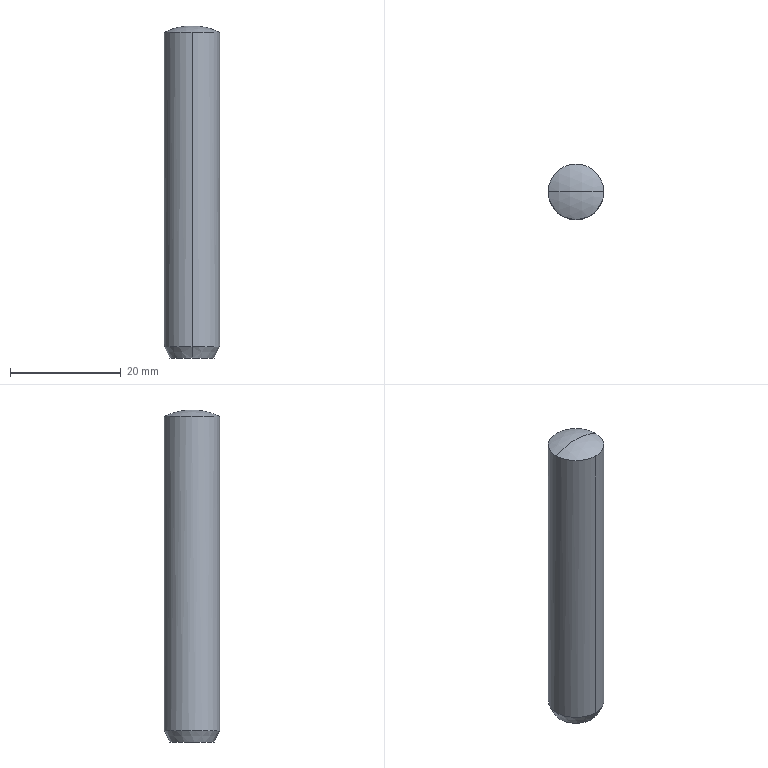Component | NX | DOWEL_PIN_10X60_2 | 1 solid | 7 faces | box 10.01 x 10.01 x 60 mm | volume 4642 mm3 | sphere 2 | cylinder 2 | cone 2 | plane 1 | commonest cylinder face diameters 10.006 x2
STEP:
#1=CARTESIAN_POINT('',(0.,0.,0.));
#2=DIRECTION('',(0.,0.,1.));
#3=DIRECTION('',(1.,0.,0.));
#4=AXIS2_PLACEMENT_3D('',#1,#2,#3);
#5=CARTESIAN_POINT('',(263.343,64.989,375.));
#6=VERTEX_POINT('',#5);
#7=CARTESIAN_POINT('',(253.337,64.989,375.));
#8=VERTEX_POINT('',#7);
#9=CARTESIAN_POINT('',(258.34,64.989,365.171));
#10=DIRECTION('',(0.,-1.,-0.));
#11=DIRECTION('',(-1.,0.,0.));
#12=AXIS2_PLACEMENT_3D('',#9,#10,#11);
#13=CIRCLE('',#12,11.029);
#14=CARTESIAN_POINT('',(258.34,64.989,365.171));
#15=DIRECTION('',(-1.,0.,0.));
#16=DIRECTION('',(0.,0.,-1.));
#17=AXIS2_PLACEMENT_3D('',#14,#15,#16);
#18=SPHERICAL_SURFACE('',#17,11.029);
#19=CARTESIAN_POINT('',(3.142,-4.712));
#20=DIRECTION('',(0.,1.));
#21=VECTOR('',#20,1.);
#22=LINE('',#19,#21);
#23=(GEOMETRIC_REPRESENTATION_CONTEXT(2)PARAMETRIC_REPRESENTATION_CONTEXT()REPRESENTATION_CONTEXT('',''));
#24=DEFINITIONAL_REPRESENTATION('',(#22),#23);
#25=PCURVE('',#18,#24);
#26=CARTESIAN_POINT('',(258.34,64.989,365.171));
#27=DIRECTION('',(-1.,0.,0.));
#28=DIRECTION('',(0.,0.,-1.));
#29=AXIS2_PLACEMENT_3D('',#26,#27,#28);
#30=SPHERICAL_SURFACE('',#29,11.029);
#31=CARTESIAN_POINT('',(3.142,-4.712));
#32=DIRECTION('',(0.,1.));
#33=VECTOR('',#32,1.);
#34=LINE('',#31,#33);
#35=(GEOMETRIC_REPRESENTATION_CONTEXT(2)PARAMETRIC_REPRESENTATION_CONTEXT()REPRESENTATION_CONTEXT('',''));
#36=DEFINITIONAL_REPRESENTATION('',(#34),#35);
#37=PCURVE('',#30,#36);
#38=SURFACE_CURVE('',#13,(#25,#37),.PCURVE_S1.);
#39=EDGE_CURVE('',#6,#8,#38,.T.);
#40=ORIENTED_EDGE('',*,*,#39,.F.);
#41=CARTESIAN_POINT('',(258.34,69.992,375.));
#42=VERTEX_POINT('',#41);
#43=CARTESIAN_POINT('',(258.34,64.989,375.));
#44=DIRECTION('',(0.,0.,1.));
#45=DIRECTION('',(0.,1.,0.));
#46=AXIS2_PLACEMENT_3D('',#43,#44,#45);
#47=CIRCLE('',#46,5.003);
#48=CARTESIAN_POINT('',(3.142,-0.4708));
#49=CARTESIAN_POINT('',(3.154,-0.4708));
#50=CARTESIAN_POINT('',(3.178,-0.47));
#51=CARTESIAN_POINT('',(3.214,-0.4661));
#52=CARTESIAN_POINT('',(3.25,-0.4596));
#53=CARTESIAN_POINT('',(3.284,-0.4507));
#54=CARTESIAN_POINT('',(3.318,-0.4394));
#55=CARTESIAN_POINT('',(3.35,-0.4257));
#56=CARTESIAN_POINT('',(3.381,-0.4098));
#57=CARTESIAN_POINT('',(3.41,-0.3919));
#58=CARTESIAN_POINT('',(3.438,-0.3719));
#59=CARTESIAN_POINT('',(3.464,-0.3502));
#60=CARTESIAN_POINT('',(3.487,-0.3268));
#61=CARTESIAN_POINT('',(3.509,-0.3018));
#62=CARTESIAN_POINT('',(3.529,-0.2755));
#63=CARTESIAN_POINT('',(3.547,-0.248));
#64=CARTESIAN_POINT('',(3.562,-0.2193));
#65=CARTESIAN_POINT('',(3.576,-0.1897));
#66=CARTESIAN_POINT('',(3.587,-0.1593));
#67=CARTESIAN_POINT('',(3.596,-0.1282));
#68=CARTESIAN_POINT('',(3.603,-0.09664));
#69=CARTESIAN_POINT('',(3.609,-0.06464));
#70=CARTESIAN_POINT('',(3.612,-0.03239));
#71=CARTESIAN_POINT('',(3.612,-0.0108));
#72=CARTESIAN_POINT('',(3.612,0.));
#73=B_SPLINE_CURVE_WITH_KNOTS('',3,(#48,#49,#50,#51,#52,#53,#54,#55,#56,#57,#58,#59,#60,#61,#62,#63,#64,#65,#66,#67,#68,#69,#70,#71,#72),.UNSPECIFIED.,.F.,.F.,(4,1,1,1,1,1,1,1,1,1,1,1,1,1,1,1,1,1,1,1,1,1,4),(4.712,4.784,4.855,4.927,4.998,5.069,5.141,5.212,5.284,5.355,5.426,5.498,5.569,5.641,5.712,5.783,5.855,5.926,5.998,6.069,6.14,6.212,6.283),.QUASI_UNIFORM_KNOTS.);
#74=(GEOMETRIC_REPRESENTATION_CONTEXT(2)PARAMETRIC_REPRESENTATION_CONTEXT()REPRESENTATION_CONTEXT('',''));
#75=DEFINITIONAL_REPRESENTATION('',(#73),#74);
#76=PCURVE('',#18,#75);
#77=CARTESIAN_POINT('',(258.34,64.989,336.601));
#78=DIRECTION('',(0.,0.,1.));
#79=DIRECTION('',(0.,-1.,0.));
#80=AXIS2_PLACEMENT_3D('',#77,#78,#79);
#81=CYLINDRICAL_SURFACE('',#80,5.003);
#82=CARTESIAN_POINT('',(-3.142,38.399));
#83=DIRECTION('',(1.,0.));
#84=VECTOR('',#83,1.);
#85=LINE('',#82,#84);
#86=(GEOMETRIC_REPRESENTATION_CONTEXT(2)PARAMETRIC_REPRESENTATION_CONTEXT()REPRESENTATION_CONTEXT('',''));
#87=DEFINITIONAL_REPRESENTATION('',(#85),#86);
#88=PCURVE('',#81,#87);
#89=SURFACE_CURVE('',#47,(#76,#88),.PCURVE_S1.);
#90=EDGE_CURVE('',#6,#42,#89,.T.);
#91=ORIENTED_EDGE('',*,*,#90,.T.);
#92=CARTESIAN_POINT('',(258.34,64.989,375.));
#93=DIRECTION('',(0.,0.,1.));
#94=DIRECTION('',(0.,1.,0.));
#95=AXIS2_PLACEMENT_3D('',#92,#93,#94);
#96=CIRCLE('',#95,5.003);
#97=CARTESIAN_POINT('',(3.612,0.));
#98=CARTESIAN_POINT('',(3.612,0.0108));
#99=CARTESIAN_POINT('',(3.612,0.03239));
#100=CARTESIAN_POINT('',(3.609,0.06464));
#101=CARTESIAN_POINT('',(3.603,0.09664));
#102=CARTESIAN_POINT('',(3.596,0.1282));
#103=CARTESIAN_POINT('',(3.587,0.1593));
#104=CARTESIAN_POINT('',(3.576,0.1897));
#105=CARTESIAN_POINT('',(3.562,0.2193));
#106=CARTESIAN_POINT('',(3.547,0.248));
#107=CARTESIAN_POINT('',(3.529,0.2755));
#108=CARTESIAN_POINT('',(3.509,0.3018));
#109=CARTESIAN_POINT('',(3.487,0.3268));
#110=CARTESIAN_POINT('',(3.464,0.3502));
#111=CARTESIAN_POINT('',(3.438,0.3719));
#112=CARTESIAN_POINT('',(3.41,0.3919));
#113=CARTESIAN_POINT('',(3.381,0.4098));
#114=CARTESIAN_POINT('',(3.35,0.4257));
#115=CARTESIAN_POINT('',(3.318,0.4394));
#116=CARTESIAN_POINT('',(3.284,0.4507));
#117=CARTESIAN_POINT('',(3.25,0.4596));
#118=CARTESIAN_POINT('',(3.214,0.4661));
#119=CARTESIAN_POINT('',(3.178,0.47));
#120=CARTESIAN_POINT('',(3.154,0.4708));
#121=CARTESIAN_POINT('',(3.142,0.4708));
#122=B_SPLINE_CURVE_WITH_KNOTS('',3,(#97,#98,#99,#100,#101,#102,#103,#104,#105,#106,#107,#108,#109,#110,#111,#112,#113,#114,#115,#116,#117,#118,#119,#120,#121),.UNSPECIFIED.,.F.,.F.,(4,1,1,1,1,1,1,1,1,1,1,1,1,1,1,1,1,1,1,1,1,1,4),(0.,0.0714,0.1428,0.2142,0.2856,0.357,0.4284,0.4998,0.5712,0.6426,0.714,0.7854,0.8568,0.9282,0.9996,1.071,1.142,1.214,1.285,1.357,1.428,1.499,1.571),.QUASI_UNIFORM_KNOTS.);
#123=(GEOMETRIC_REPRESENTATION_CONTEXT(2)PARAMETRIC_REPRESENTATION_CONTEXT()REPRESENTATION_CONTEXT('',''));
#124=DEFINITIONAL_REPRESENTATION('',(#122),#123);
#125=PCURVE('',#18,#124);
#126=CARTESIAN_POINT('',(258.34,64.989,336.601));
#127=DIRECTION('',(0.,0.,1.));
#128=DIRECTION('',(0.,-1.,0.));
#129=AXIS2_PLACEMENT_3D('',#126,#127,#128);
#130=CYLINDRICAL_SURFACE('',#129,5.003);
#131=CARTESIAN_POINT('',(3.142,38.399));
#132=DIRECTION('',(1.,0.));
#133=VECTOR('',#132,1.);
#134=LINE('',#131,#133);
#135=(GEOMETRIC_REPRESENTATION_CONTEXT(2)PARAMETRIC_REPRESENTATION_CONTEXT()REPRESENTATION_CONTEXT('',''));
#136=DEFINITIONAL_REPRESENTATION('',(#134),#135);
#137=PCURVE('',#130,#136);
#138=SURFACE_CURVE('',#96,(#125,#137),.PCURVE_S1.);
#139=EDGE_CURVE('',#42,#8,#138,.T.);
#140=ORIENTED_EDGE('',*,*,#139,.T.);
#141=EDGE_LOOP('',(#40,#91,#140));
#142=FACE_BOUND('',#141,.T.);
#143=ADVANCED_FACE('',(#142),#18,.T.);
#144=CARTESIAN_POINT('',(258.34,69.992,318.201));
#145=VERTEX_POINT('',#144);
#146=CARTESIAN_POINT('',(258.34,69.992,336.601));
#147=DIRECTION('',(0.,0.,1.));
#148=VECTOR('',#147,1.);
#149=LINE('',#146,#148);
#150=CARTESIAN_POINT('',(3.142,0.));
#151=DIRECTION('',(0.,1.));
#152=VECTOR('',#151,1.);
#153=LINE('',#150,#152);
#154=(GEOMETRIC_REPRESENTATION_CONTEXT(2)PARAMETRIC_REPRESENTATION_CONTEXT()REPRESENTATION_CONTEXT('',''));
#155=DEFINITIONAL_REPRESENTATION('',(#153),#154);
#156=PCURVE('',#130,#155);
#157=CARTESIAN_POINT('',(3.142,0.));
#158=DIRECTION('',(0.,1.));
#159=VECTOR('',#158,1.);
#160=LINE('',#157,#159);
#161=(GEOMETRIC_REPRESENTATION_CONTEXT(2)PARAMETRIC_REPRESENTATION_CONTEXT()REPRESENTATION_CONTEXT('',''));
#162=DEFINITIONAL_REPRESENTATION('',(#160),#161);
#163=PCURVE('',#81,#162);
#164=SURFACE_CURVE('',#149,(#156,#163),.PCURVE_S1.);
#165=EDGE_CURVE('',#145,#42,#164,.T.);
#166=ORIENTED_EDGE('',*,*,#165,.F.);
#167=CARTESIAN_POINT('',(258.34,59.986,318.201));
#168=VERTEX_POINT('',#167);
#169=CARTESIAN_POINT('',(258.34,64.989,318.201));
#170=DIRECTION('',(0.,0.,1.));
#171=DIRECTION('',(0.,1.,0.));
#172=AXIS2_PLACEMENT_3D('',#169,#170,#171);
#173=CIRCLE('',#172,5.003);
#174=CARTESIAN_POINT('',(3.142,-18.399));
#175=DIRECTION('',(1.,0.));
#176=VECTOR('',#175,1.);
#177=LINE('',#174,#176);
#178=(GEOMETRIC_REPRESENTATION_CONTEXT(2)PARAMETRIC_REPRESENTATION_CONTEXT()REPRESENTATION_CONTEXT('',''));
#179=DEFINITIONAL_REPRESENTATION('',(#177),#178);
#180=PCURVE('',#130,#179);
#181=CARTESIAN_POINT('',(258.34,64.989,317.201));
#182=DIRECTION('',(0.,0.,1.));
#183=DIRECTION('',(0.,-1.,0.));
#184=AXIS2_PLACEMENT_3D('',#181,#182,#183);
#185=CONICAL_SURFACE('',#184,4.503,0.4636);
#186=CARTESIAN_POINT('',(3.142,1.001));
#187=DIRECTION('',(1.,0.));
#188=VECTOR('',#187,1.);
#189=LINE('',#186,#188);
#190=(GEOMETRIC_REPRESENTATION_CONTEXT(2)PARAMETRIC_REPRESENTATION_CONTEXT()REPRESENTATION_CONTEXT('',''));
#191=DEFINITIONAL_REPRESENTATION('',(#189),#190);
#192=PCURVE('',#185,#191);
#193=SURFACE_CURVE('',#173,(#180,#192),.PCURVE_S1.);
#194=EDGE_CURVE('',#145,#168,#193,.T.);
#195=ORIENTED_EDGE('',*,*,#194,.T.);
#196=CARTESIAN_POINT('',(258.34,59.986,375.));
#197=VERTEX_POINT('',#196);
#198=CARTESIAN_POINT('',(258.34,59.986,336.601));
#199=DIRECTION('',(0.,0.,-1.));
#200=VECTOR('',#199,1.);
#201=LINE('',#198,#200);
#202=CARTESIAN_POINT('',(6.283,0.));
#203=DIRECTION('',(0.,-1.));
#204=VECTOR('',#203,1.);
#205=LINE('',#202,#204);
#206=(GEOMETRIC_REPRESENTATION_CONTEXT(2)PARAMETRIC_REPRESENTATION_CONTEXT()REPRESENTATION_CONTEXT('',''));
#207=DEFINITIONAL_REPRESENTATION('',(#205),#206);
#208=PCURVE('',#130,#207);
#209=CARTESIAN_POINT('',(0.,0.));
#210=DIRECTION('',(0.,-1.));
#211=VECTOR('',#210,1.);
#212=LINE('',#209,#211);
#213=(GEOMETRIC_REPRESENTATION_CONTEXT(2)PARAMETRIC_REPRESENTATION_CONTEXT()REPRESENTATION_CONTEXT('',''));
#214=DEFINITIONAL_REPRESENTATION('',(#212),#213);
#215=PCURVE('',#81,#214);
#216=SURFACE_CURVE('',#201,(#208,#215),.PCURVE_S1.);
#217=EDGE_CURVE('',#197,#168,#216,.T.);
#218=ORIENTED_EDGE('',*,*,#217,.F.);
#219=CARTESIAN_POINT('',(258.34,64.989,375.));
#220=DIRECTION('',(0.,0.,1.));
#221=DIRECTION('',(0.,1.,0.));
#222=AXIS2_PLACEMENT_3D('',#219,#220,#221);
#223=CIRCLE('',#222,5.003);
#224=CARTESIAN_POINT('',(3.142,38.399));
#225=DIRECTION('',(1.,0.));
#226=VECTOR('',#225,1.);
#227=LINE('',#224,#226);
#228=(GEOMETRIC_REPRESENTATION_CONTEXT(2)PARAMETRIC_REPRESENTATION_CONTEXT()REPRESENTATION_CONTEXT('',''));
#229=DEFINITIONAL_REPRESENTATION('',(#227),#228);
#230=PCURVE('',#130,#229);
#231=CARTESIAN_POINT('',(3.142,0.4708));
#232=CARTESIAN_POINT('',(3.129,0.4708));
#233=CARTESIAN_POINT('',(3.105,0.47));
#234=CARTESIAN_POINT('',(3.069,0.4661));
#235=CARTESIAN_POINT('',(3.034,0.4596));
#236=CARTESIAN_POINT('',(2.999,0.4507));
#237=CARTESIAN_POINT('',(2.965,0.4394));
#238=CARTESIAN_POINT('',(2.933,0.4257));
#239=CARTESIAN_POINT('',(2.902,0.4098));
#240=CARTESIAN_POINT('',(2.873,0.3919));
#241=CARTESIAN_POINT('',(2.845,0.3719));
#242=CARTESIAN_POINT('',(2.82,0.3502));
#243=CARTESIAN_POINT('',(2.796,0.3268));
#244=CARTESIAN_POINT('',(2.774,0.3018));
#245=CARTESIAN_POINT('',(2.754,0.2755));
#246=CARTESIAN_POINT('',(2.737,0.248));
#247=CARTESIAN_POINT('',(2.721,0.2193));
#248=CARTESIAN_POINT('',(2.708,0.1897));
#249=CARTESIAN_POINT('',(2.696,0.1593));
#250=CARTESIAN_POINT('',(2.687,0.1282));
#251=CARTESIAN_POINT('',(2.68,0.09664));
#252=CARTESIAN_POINT('',(2.675,0.06464));
#253=CARTESIAN_POINT('',(2.671,0.03239));
#254=CARTESIAN_POINT('',(2.671,0.0108));
#255=CARTESIAN_POINT('',(2.671,0.));
#256=B_SPLINE_CURVE_WITH_KNOTS('',3,(#231,#232,#233,#234,#235,#236,#237,#238,#239,#240,#241,#242,#243,#244,#245,#246,#247,#248,#249,#250,#251,#252,#253,#254,#255),.UNSPECIFIED.,.F.,.F.,(4,1,1,1,1,1,1,1,1,1,1,1,1,1,1,1,1,1,1,1,1,1,4),(1.571,1.642,1.714,1.785,1.856,1.928,1.999,2.071,2.142,2.213,2.285,2.356,2.428,2.499,2.57,2.642,2.713,2.785,2.856,2.927,2.999,3.07,3.142),.QUASI_UNIFORM_KNOTS.);
#257=(GEOMETRIC_REPRESENTATION_CONTEXT(2)PARAMETRIC_REPRESENTATION_CONTEXT()REPRESENTATION_CONTEXT('',''));
#258=DEFINITIONAL_REPRESENTATION('',(#256),#257);
#259=PCURVE('',#30,#258);
#260=SURFACE_CURVE('',#223,(#230,#259),.PCURVE_S1.);
#261=EDGE_CURVE('',#8,#197,#260,.T.);
#262=ORIENTED_EDGE('',*,*,#261,.F.);
#263=ORIENTED_EDGE('',*,*,#139,.F.);
#264=EDGE_LOOP('',(#166,#195,#218,#262,#263));
#265=FACE_BOUND('',#264,.T.);
#266=ADVANCED_FACE('',(#265),#130,.T.);
#267=CARTESIAN_POINT('',(258.34,68.991,316.2));
#268=VERTEX_POINT('',#267);
#269=CARTESIAN_POINT('',(258.34,69.491,317.201));
#270=DIRECTION('',(0.,0.4472,0.8944));
#271=VECTOR('',#270,1.);
#272=LINE('',#269,#271);
#273=CARTESIAN_POINT('',(3.142,-0.));
#274=DIRECTION('',(0.,1.));
#275=VECTOR('',#274,1.);
#276=LINE('',#273,#275);
#277=(GEOMETRIC_REPRESENTATION_CONTEXT(2)PARAMETRIC_REPRESENTATION_CONTEXT()REPRESENTATION_CONTEXT('',''));
#278=DEFINITIONAL_REPRESENTATION('',(#276),#277);
#279=PCURVE('',#185,#278);
#280=CARTESIAN_POINT('',(258.34,64.989,317.201));
#281=DIRECTION('',(0.,0.,1.));
#282=DIRECTION('',(0.,-1.,0.));
#283=AXIS2_PLACEMENT_3D('',#280,#281,#282);
#284=CONICAL_SURFACE('',#283,4.503,0.4636);
#285=CARTESIAN_POINT('',(3.142,-0.));
#286=DIRECTION('',(0.,1.));
#287=VECTOR('',#286,1.);
#288=LINE('',#285,#287);
#289=(GEOMETRIC_REPRESENTATION_CONTEXT(2)PARAMETRIC_REPRESENTATION_CONTEXT()REPRESENTATION_CONTEXT('',''));
#290=DEFINITIONAL_REPRESENTATION('',(#288),#289);
#291=PCURVE('',#284,#290);
#292=SURFACE_CURVE('',#272,(#279,#291),.PCURVE_S1.);
#293=EDGE_CURVE('',#268,#145,#292,.T.);
#294=ORIENTED_EDGE('',*,*,#293,.F.);
#295=CARTESIAN_POINT('',(258.34,60.986,316.2));
#296=VERTEX_POINT('',#295);
#297=CARTESIAN_POINT('',(258.34,64.989,316.2));
#298=DIRECTION('',(0.,0.,1.));
#299=DIRECTION('',(0.,1.,0.));
#300=AXIS2_PLACEMENT_3D('',#297,#298,#299);
#301=CIRCLE('',#300,4.002);
#302=CARTESIAN_POINT('',(3.142,-1.001));
#303=DIRECTION('',(1.,0.));
#304=VECTOR('',#303,1.);
#305=LINE('',#302,#304);
#306=(GEOMETRIC_REPRESENTATION_CONTEXT(2)PARAMETRIC_REPRESENTATION_CONTEXT()REPRESENTATION_CONTEXT('',''));
#307=DEFINITIONAL_REPRESENTATION('',(#305),#306);
#308=PCURVE('',#185,#307);
#309=CARTESIAN_POINT('',(258.34,66.99,316.2));
#310=DIRECTION('',(0.,-0.,-1.));
#311=DIRECTION('',(0.,1.,-0.));
#312=AXIS2_PLACEMENT_3D('',#309,#310,#311);
#313=PLANE('',#312);
#314=CARTESIAN_POINT('',(2.001,0.));
#315=CARTESIAN_POINT('',(2.001,-6.932));
#316=CARTESIAN_POINT('',(-4.002,-3.466));
#317=CARTESIAN_POINT('',(-10.006,-0.));
#318=CARTESIAN_POINT('',(-4.002,3.466));
#319=CARTESIAN_POINT('',(2.001,6.932));
#320=CARTESIAN_POINT('',(2.001,0.));
#321=(BOUNDED_CURVE()B_SPLINE_CURVE(2,(#314,#315,#316,#317,#318,#319,#320),.UNSPECIFIED.,.T.,.F.)B_SPLINE_CURVE_WITH_KNOTS((1,2,2,2,2,1),(-2.094,0.,2.094,4.189,6.283,8.378),.UNSPECIFIED.)CURVE()GEOMETRIC_REPRESENTATION_ITEM()RATIONAL_B_SPLINE_CURVE((1.,0.5,1.,0.5,1.,0.5,1.))REPRESENTATION_ITEM(''));
#322=(GEOMETRIC_REPRESENTATION_CONTEXT(2)PARAMETRIC_REPRESENTATION_CONTEXT()REPRESENTATION_CONTEXT('',''));
#323=DEFINITIONAL_REPRESENTATION('',(#321),#322);
#324=PCURVE('',#313,#323);
#325=SURFACE_CURVE('',#301,(#308,#324),.PCURVE_S1.);
#326=EDGE_CURVE('',#268,#296,#325,.T.);
#327=ORIENTED_EDGE('',*,*,#326,.T.);
#328=CARTESIAN_POINT('',(258.34,60.486,317.201));
#329=DIRECTION('',(0.,0.4472,-0.8944));
#330=VECTOR('',#329,1.);
#331=LINE('',#328,#330);
#332=CARTESIAN_POINT('',(6.283,-0.));
#333=DIRECTION('',(0.,-1.));
#334=VECTOR('',#333,1.);
#335=LINE('',#332,#334);
#336=(GEOMETRIC_REPRESENTATION_CONTEXT(2)PARAMETRIC_REPRESENTATION_CONTEXT()REPRESENTATION_CONTEXT('',''));
#337=DEFINITIONAL_REPRESENTATION('',(#335),#336);
#338=PCURVE('',#185,#337);
#339=CARTESIAN_POINT('',(0.,-0.));
#340=DIRECTION('',(0.,-1.));
#341=VECTOR('',#340,1.);
#342=LINE('',#339,#341);
#343=(GEOMETRIC_REPRESENTATION_CONTEXT(2)PARAMETRIC_REPRESENTATION_CONTEXT()REPRESENTATION_CONTEXT('',''));
#344=DEFINITIONAL_REPRESENTATION('',(#342),#343);
#345=PCURVE('',#284,#344);
#346=SURFACE_CURVE('',#331,(#338,#345),.PCURVE_S1.);
#347=EDGE_CURVE('',#168,#296,#346,.T.);
#348=ORIENTED_EDGE('',*,*,#347,.F.);
#349=ORIENTED_EDGE('',*,*,#194,.F.);
#350=EDGE_LOOP('',(#294,#327,#348,#349));
#351=FACE_BOUND('',#350,.T.);
#352=ADVANCED_FACE('',(#351),#185,.T.);
#353=ORIENTED_EDGE('',*,*,#293,.T.);
#354=CARTESIAN_POINT('',(258.34,64.989,318.201));
#355=DIRECTION('',(0.,0.,1.));
#356=DIRECTION('',(0.,1.,0.));
#357=AXIS2_PLACEMENT_3D('',#354,#355,#356);
#358=CIRCLE('',#357,5.003);
#359=CARTESIAN_POINT('',(-3.142,1.001));
#360=DIRECTION('',(1.,0.));
#361=VECTOR('',#360,1.);
#362=LINE('',#359,#361);
#363=(GEOMETRIC_REPRESENTATION_CONTEXT(2)PARAMETRIC_REPRESENTATION_CONTEXT()REPRESENTATION_CONTEXT('',''));
#364=DEFINITIONAL_REPRESENTATION('',(#362),#363);
#365=PCURVE('',#284,#364);
#366=CARTESIAN_POINT('',(-3.142,-18.399));
#367=DIRECTION('',(1.,0.));
#368=VECTOR('',#367,1.);
#369=LINE('',#366,#368);
#370=(GEOMETRIC_REPRESENTATION_CONTEXT(2)PARAMETRIC_REPRESENTATION_CONTEXT()REPRESENTATION_CONTEXT('',''));
#371=DEFINITIONAL_REPRESENTATION('',(#369),#370);
#372=PCURVE('',#81,#371);
#373=SURFACE_CURVE('',#358,(#365,#372),.PCURVE_S1.);
#374=EDGE_CURVE('',#168,#145,#373,.T.);
#375=ORIENTED_EDGE('',*,*,#374,.F.);
#376=ORIENTED_EDGE('',*,*,#347,.T.);
#377=CARTESIAN_POINT('',(258.34,64.989,316.2));
#378=DIRECTION('',(0.,0.,1.));
#379=DIRECTION('',(0.,1.,0.));
#380=AXIS2_PLACEMENT_3D('',#377,#378,#379);
#381=CIRCLE('',#380,4.002);
#382=CARTESIAN_POINT('',(-3.142,-1.001));
#383=DIRECTION('',(1.,-0.));
#384=VECTOR('',#383,1.);
#385=LINE('',#382,#384);
#386=(GEOMETRIC_REPRESENTATION_CONTEXT(2)PARAMETRIC_REPRESENTATION_CONTEXT()REPRESENTATION_CONTEXT('',''));
#387=DEFINITIONAL_REPRESENTATION('',(#385),#386);
#388=PCURVE('',#284,#387);
#389=CARTESIAN_POINT('',(2.001,0.));
#390=CARTESIAN_POINT('',(2.001,-6.932));
#391=CARTESIAN_POINT('',(-4.002,-3.466));
#392=CARTESIAN_POINT('',(-10.006,-0.));
#393=CARTESIAN_POINT('',(-4.002,3.466));
#394=CARTESIAN_POINT('',(2.001,6.932));
#395=CARTESIAN_POINT('',(2.001,0.));
#396=(BOUNDED_CURVE()B_SPLINE_CURVE(2,(#389,#390,#391,#392,#393,#394,#395),.UNSPECIFIED.,.T.,.F.)B_SPLINE_CURVE_WITH_KNOTS((1,2,2,2,2,1),(-2.094,0.,2.094,4.189,6.283,8.378),.UNSPECIFIED.)CURVE()GEOMETRIC_REPRESENTATION_ITEM()RATIONAL_B_SPLINE_CURVE((1.,0.5,1.,0.5,1.,0.5,1.))REPRESENTATION_ITEM(''));
#397=(GEOMETRIC_REPRESENTATION_CONTEXT(2)PARAMETRIC_REPRESENTATION_CONTEXT()REPRESENTATION_CONTEXT('',''));
#398=DEFINITIONAL_REPRESENTATION('',(#396),#397);
#399=PCURVE('',#313,#398);
#400=SURFACE_CURVE('',#381,(#388,#399),.PCURVE_S1.);
#401=EDGE_CURVE('',#296,#268,#400,.T.);
#402=ORIENTED_EDGE('',*,*,#401,.T.);
#403=EDGE_LOOP('',(#353,#375,#376,#402));
#404=FACE_BOUND('',#403,.T.);
#405=ADVANCED_FACE('',(#404),#284,.T.);
#406=ORIENTED_EDGE('',*,*,#165,.T.);
#407=ORIENTED_EDGE('',*,*,#90,.F.);
#408=CARTESIAN_POINT('',(258.34,64.989,375.));
#409=DIRECTION('',(0.,0.,1.));
#410=DIRECTION('',(0.,1.,0.));
#411=AXIS2_PLACEMENT_3D('',#408,#409,#410);
#412=CIRCLE('',#411,5.003);
#413=CARTESIAN_POINT('',(-3.142,38.399));
#414=DIRECTION('',(1.,0.));
#415=VECTOR('',#414,1.);
#416=LINE('',#413,#415);
#417=(GEOMETRIC_REPRESENTATION_CONTEXT(2)PARAMETRIC_REPRESENTATION_CONTEXT()REPRESENTATION_CONTEXT('',''));
#418=DEFINITIONAL_REPRESENTATION('',(#416),#417);
#419=PCURVE('',#81,#418);
#420=CARTESIAN_POINT('',(2.671,0.));
#421=CARTESIAN_POINT('',(2.671,-0.0108));
#422=CARTESIAN_POINT('',(2.671,-0.03239));
#423=CARTESIAN_POINT('',(2.675,-0.06464));
#424=CARTESIAN_POINT('',(2.68,-0.09664));
#425=CARTESIAN_POINT('',(2.687,-0.1282));
#426=CARTESIAN_POINT('',(2.696,-0.1593));
#427=CARTESIAN_POINT('',(2.708,-0.1897));
#428=CARTESIAN_POINT('',(2.721,-0.2193));
#429=CARTESIAN_POINT('',(2.737,-0.248));
#430=CARTESIAN_POINT('',(2.754,-0.2755));
#431=CARTESIAN_POINT('',(2.774,-0.3018));
#432=CARTESIAN_POINT('',(2.796,-0.3268));
#433=CARTESIAN_POINT('',(2.82,-0.3502));
#434=CARTESIAN_POINT('',(2.845,-0.3719));
#435=CARTESIAN_POINT('',(2.873,-0.3919));
#436=CARTESIAN_POINT('',(2.902,-0.4098));
#437=CARTESIAN_POINT('',(2.933,-0.4257));
#438=CARTESIAN_POINT('',(2.965,-0.4394));
#439=CARTESIAN_POINT('',(2.999,-0.4507));
#440=CARTESIAN_POINT('',(3.034,-0.4596));
#441=CARTESIAN_POINT('',(3.069,-0.4661));
#442=CARTESIAN_POINT('',(3.105,-0.47));
#443=CARTESIAN_POINT('',(3.129,-0.4708));
#444=CARTESIAN_POINT('',(3.142,-0.4708));
#445=B_SPLINE_CURVE_WITH_KNOTS('',3,(#420,#421,#422,#423,#424,#425,#426,#427,#428,#429,#430,#431,#432,#433,#434,#435,#436,#437,#438,#439,#440,#441,#442,#443,#444),.UNSPECIFIED.,.F.,.F.,(4,1,1,1,1,1,1,1,1,1,1,1,1,1,1,1,1,1,1,1,1,1,4),(3.142,3.213,3.284,3.356,3.427,3.499,3.57,3.641,3.713,3.784,3.856,3.927,3.998,4.07,4.141,4.213,4.284,4.355,4.427,4.498,4.57,4.641,4.712),.QUASI_UNIFORM_KNOTS.);
#446=(GEOMETRIC_REPRESENTATION_CONTEXT(2)PARAMETRIC_REPRESENTATION_CONTEXT()REPRESENTATION_CONTEXT('',''));
#447=DEFINITIONAL_REPRESENTATION('',(#445),#446);
#448=PCURVE('',#30,#447);
#449=SURFACE_CURVE('',#412,(#419,#448),.PCURVE_S1.);
#450=EDGE_CURVE('',#197,#6,#449,.T.);
#451=ORIENTED_EDGE('',*,*,#450,.F.);
#452=ORIENTED_EDGE('',*,*,#217,.T.);
#453=ORIENTED_EDGE('',*,*,#374,.T.);
#454=EDGE_LOOP('',(#406,#407,#451,#452,#453));
#455=FACE_BOUND('',#454,.T.);
#456=ADVANCED_FACE('',(#455),#81,.T.);
#457=ORIENTED_EDGE('',*,*,#39,.T.);
#458=ORIENTED_EDGE('',*,*,#261,.T.);
#459=ORIENTED_EDGE('',*,*,#450,.T.);
#460=EDGE_LOOP('',(#457,#458,#459));
#461=FACE_BOUND('',#460,.T.);
#462=ADVANCED_FACE('',(#461),#30,.T.);
#463=ORIENTED_EDGE('',*,*,#326,.F.);
#464=ORIENTED_EDGE('',*,*,#401,.F.);
#465=EDGE_LOOP('',(#463,#464));
#466=FACE_BOUND('',#465,.T.);
#467=ADVANCED_FACE('',(#466),#313,.T.);
#468=CLOSED_SHELL('',(#143,#266,#352,#405,#456,#462,#467));
#469=MANIFOLD_SOLID_BREP('',#468);
#470=(LENGTH_UNIT()NAMED_UNIT(*)SI_UNIT(.MILLI.,.METRE.));
#471=UNCERTAINTY_MEASURE_WITH_UNIT(LENGTH_MEASURE(0.0000001),#470,'','');
#472=(NAMED_UNIT(*)PLANE_ANGLE_UNIT()SI_UNIT($,.RADIAN.));
#473=(NAMED_UNIT(*)SI_UNIT($,.STERADIAN.)SOLID_ANGLE_UNIT());
#474=(GEOMETRIC_REPRESENTATION_CONTEXT(3)GLOBAL_UNCERTAINTY_ASSIGNED_CONTEXT((#471))GLOBAL_UNIT_ASSIGNED_CONTEXT((#470,#472,#473))REPRESENTATION_CONTEXT('',''));
#475=ADVANCED_BREP_SHAPE_REPRESENTATION('',(#4,#469),#474);